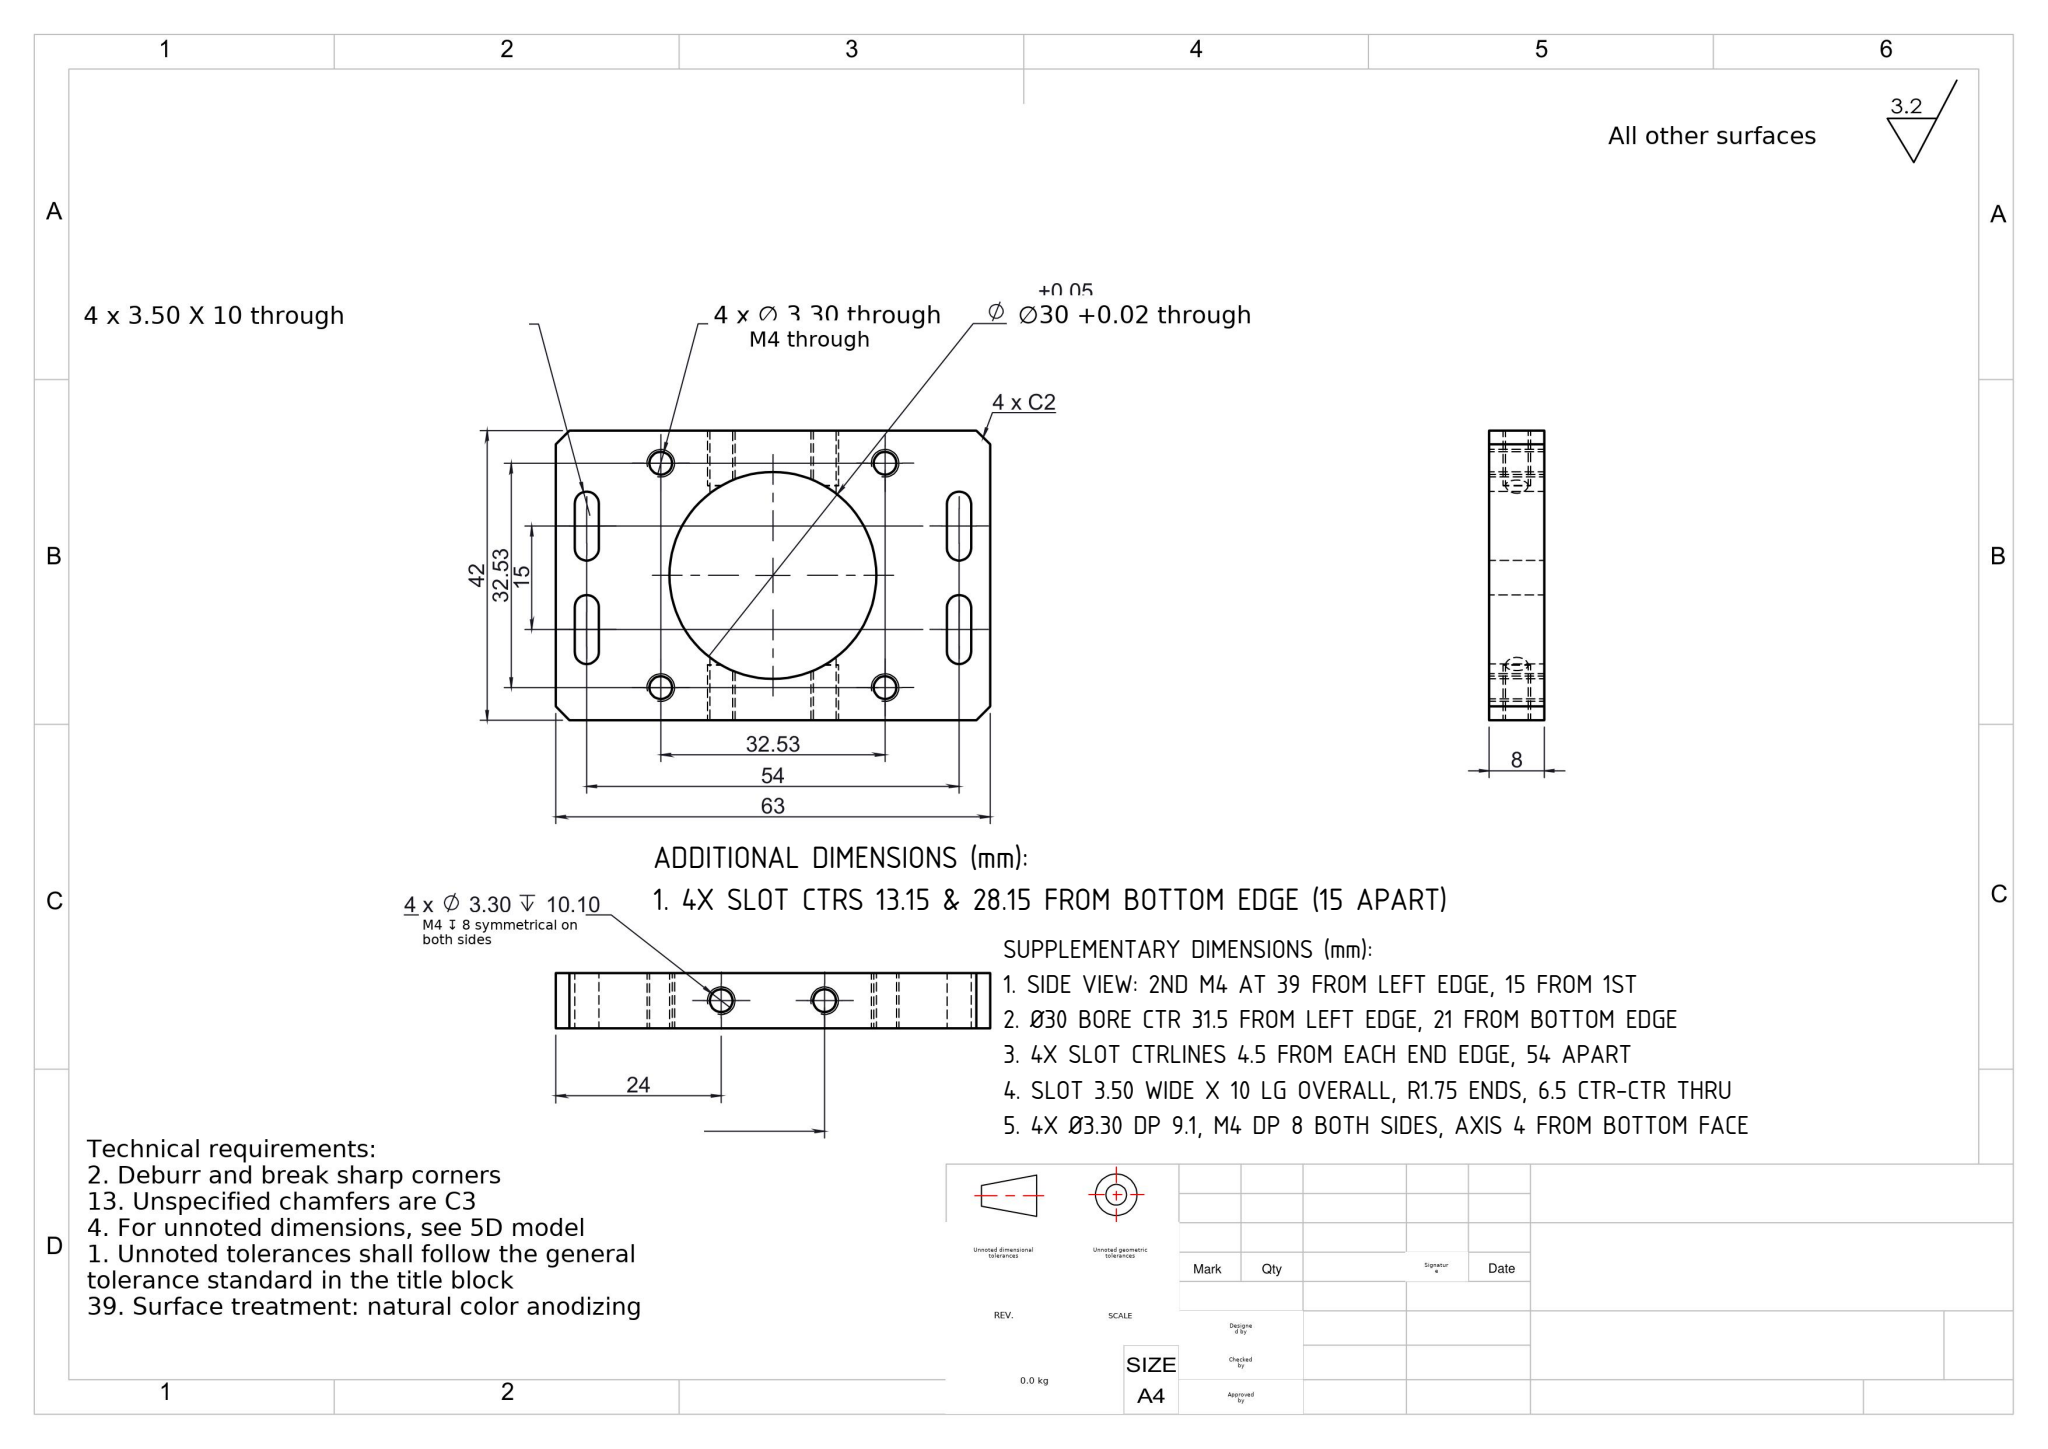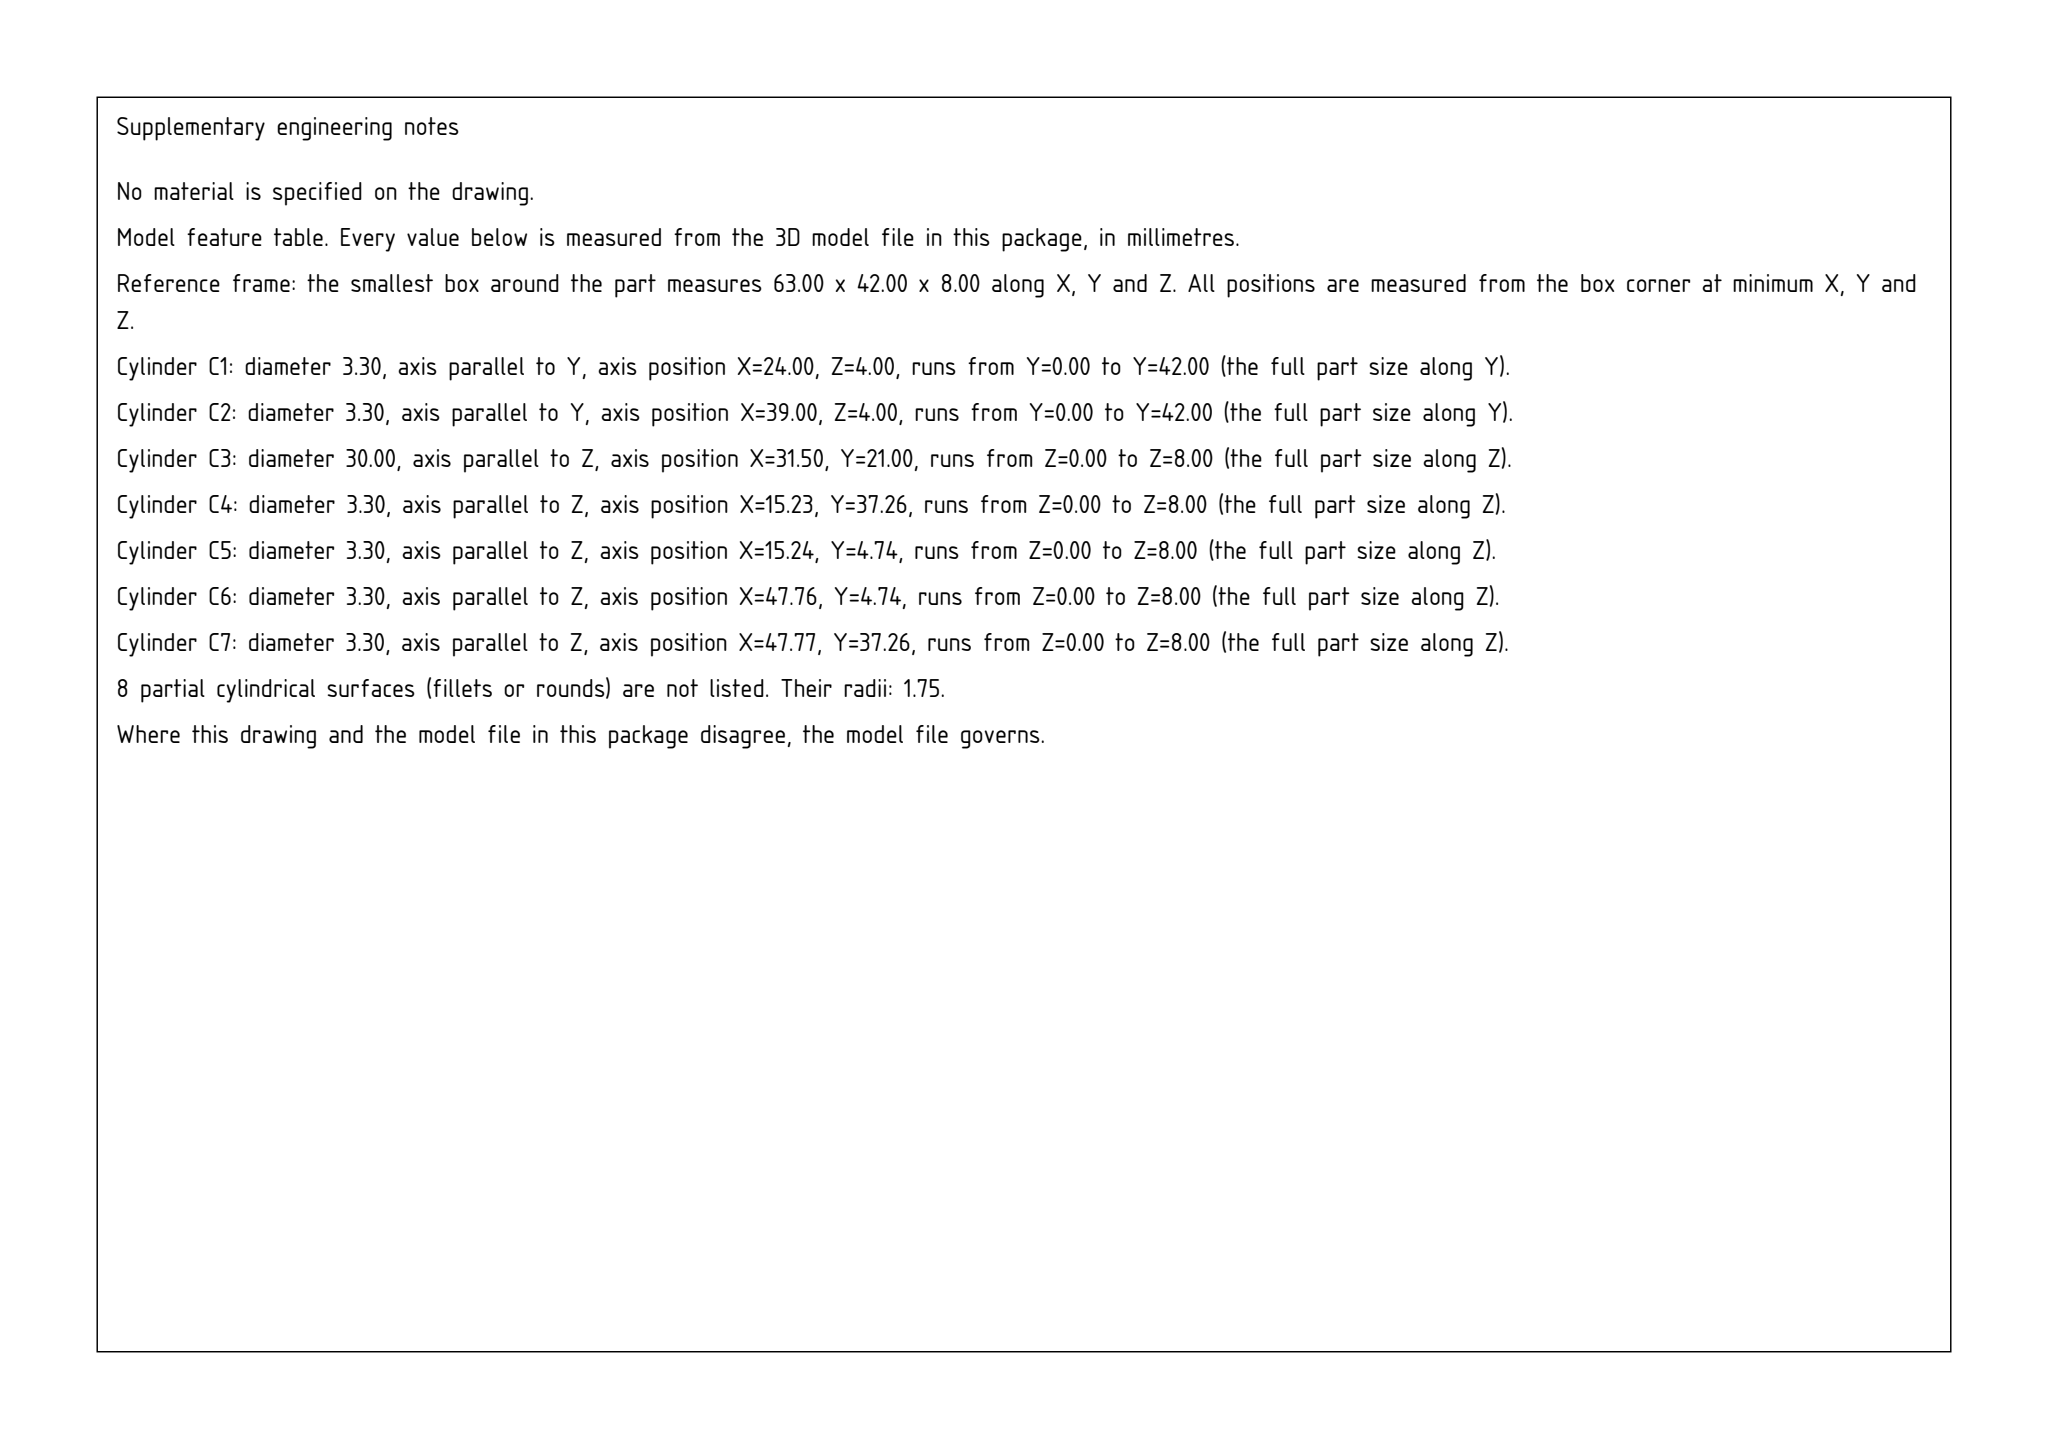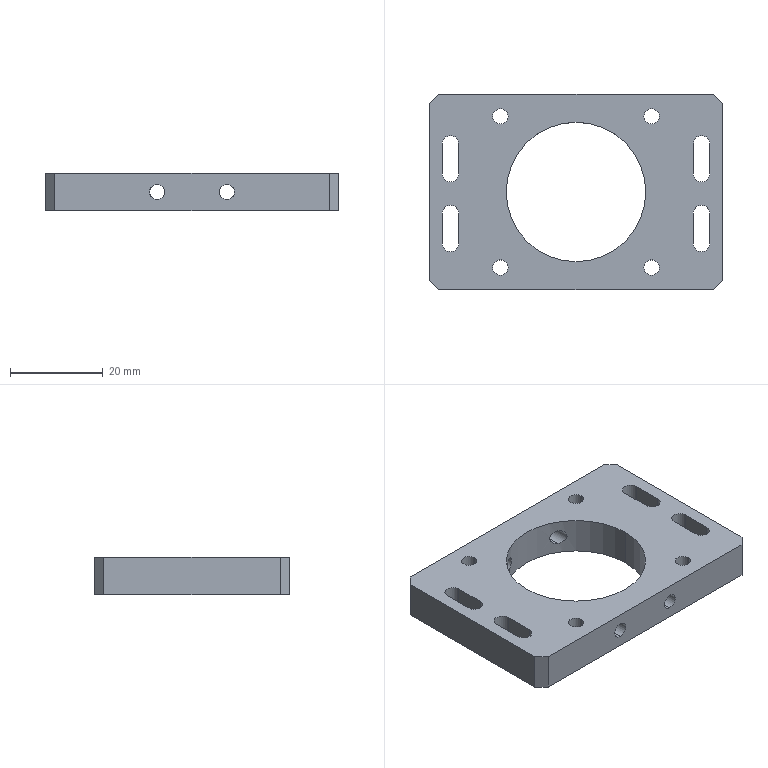Part | SolidWorks | mm | 1 solid | 44 faces | box 63 x 42 x 8 mm | volume 13864 mm3 | cylinder 26 | plane 18 | commonest cylinder face diameters 3.3 x16 3.5 x8 30 x2